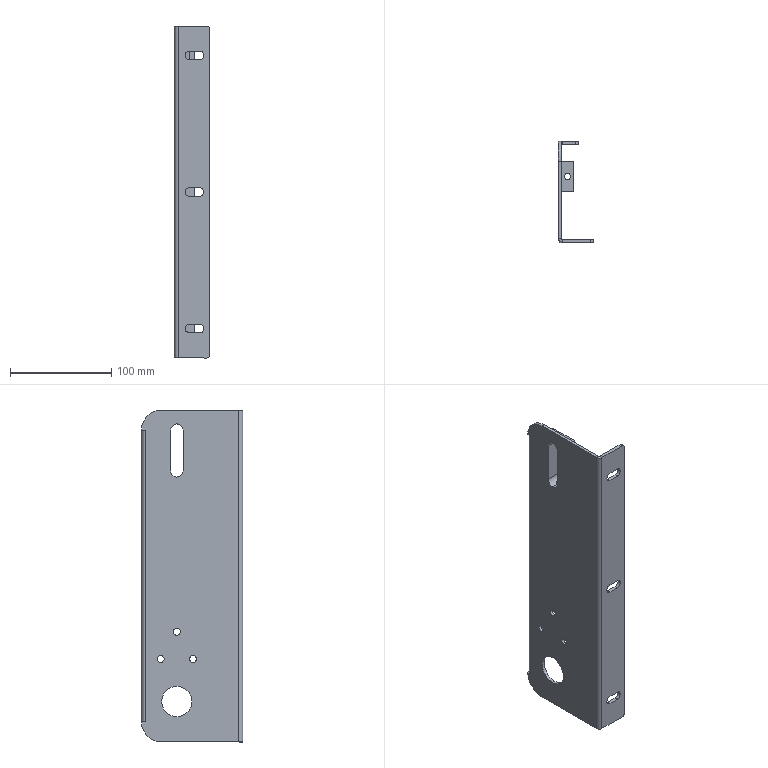Component | SolidWorks | CCD04BearingSupportPlateA-1 | 1 solid | 73 faces | volume 150272 mm3 | cylinder 40 | plane 33 | commonest cylinder face diameters 8.5 x9 5 x6 6.8 x6 6.2 x4 6 x4 12.5 x3 30 x2 7.473 x2